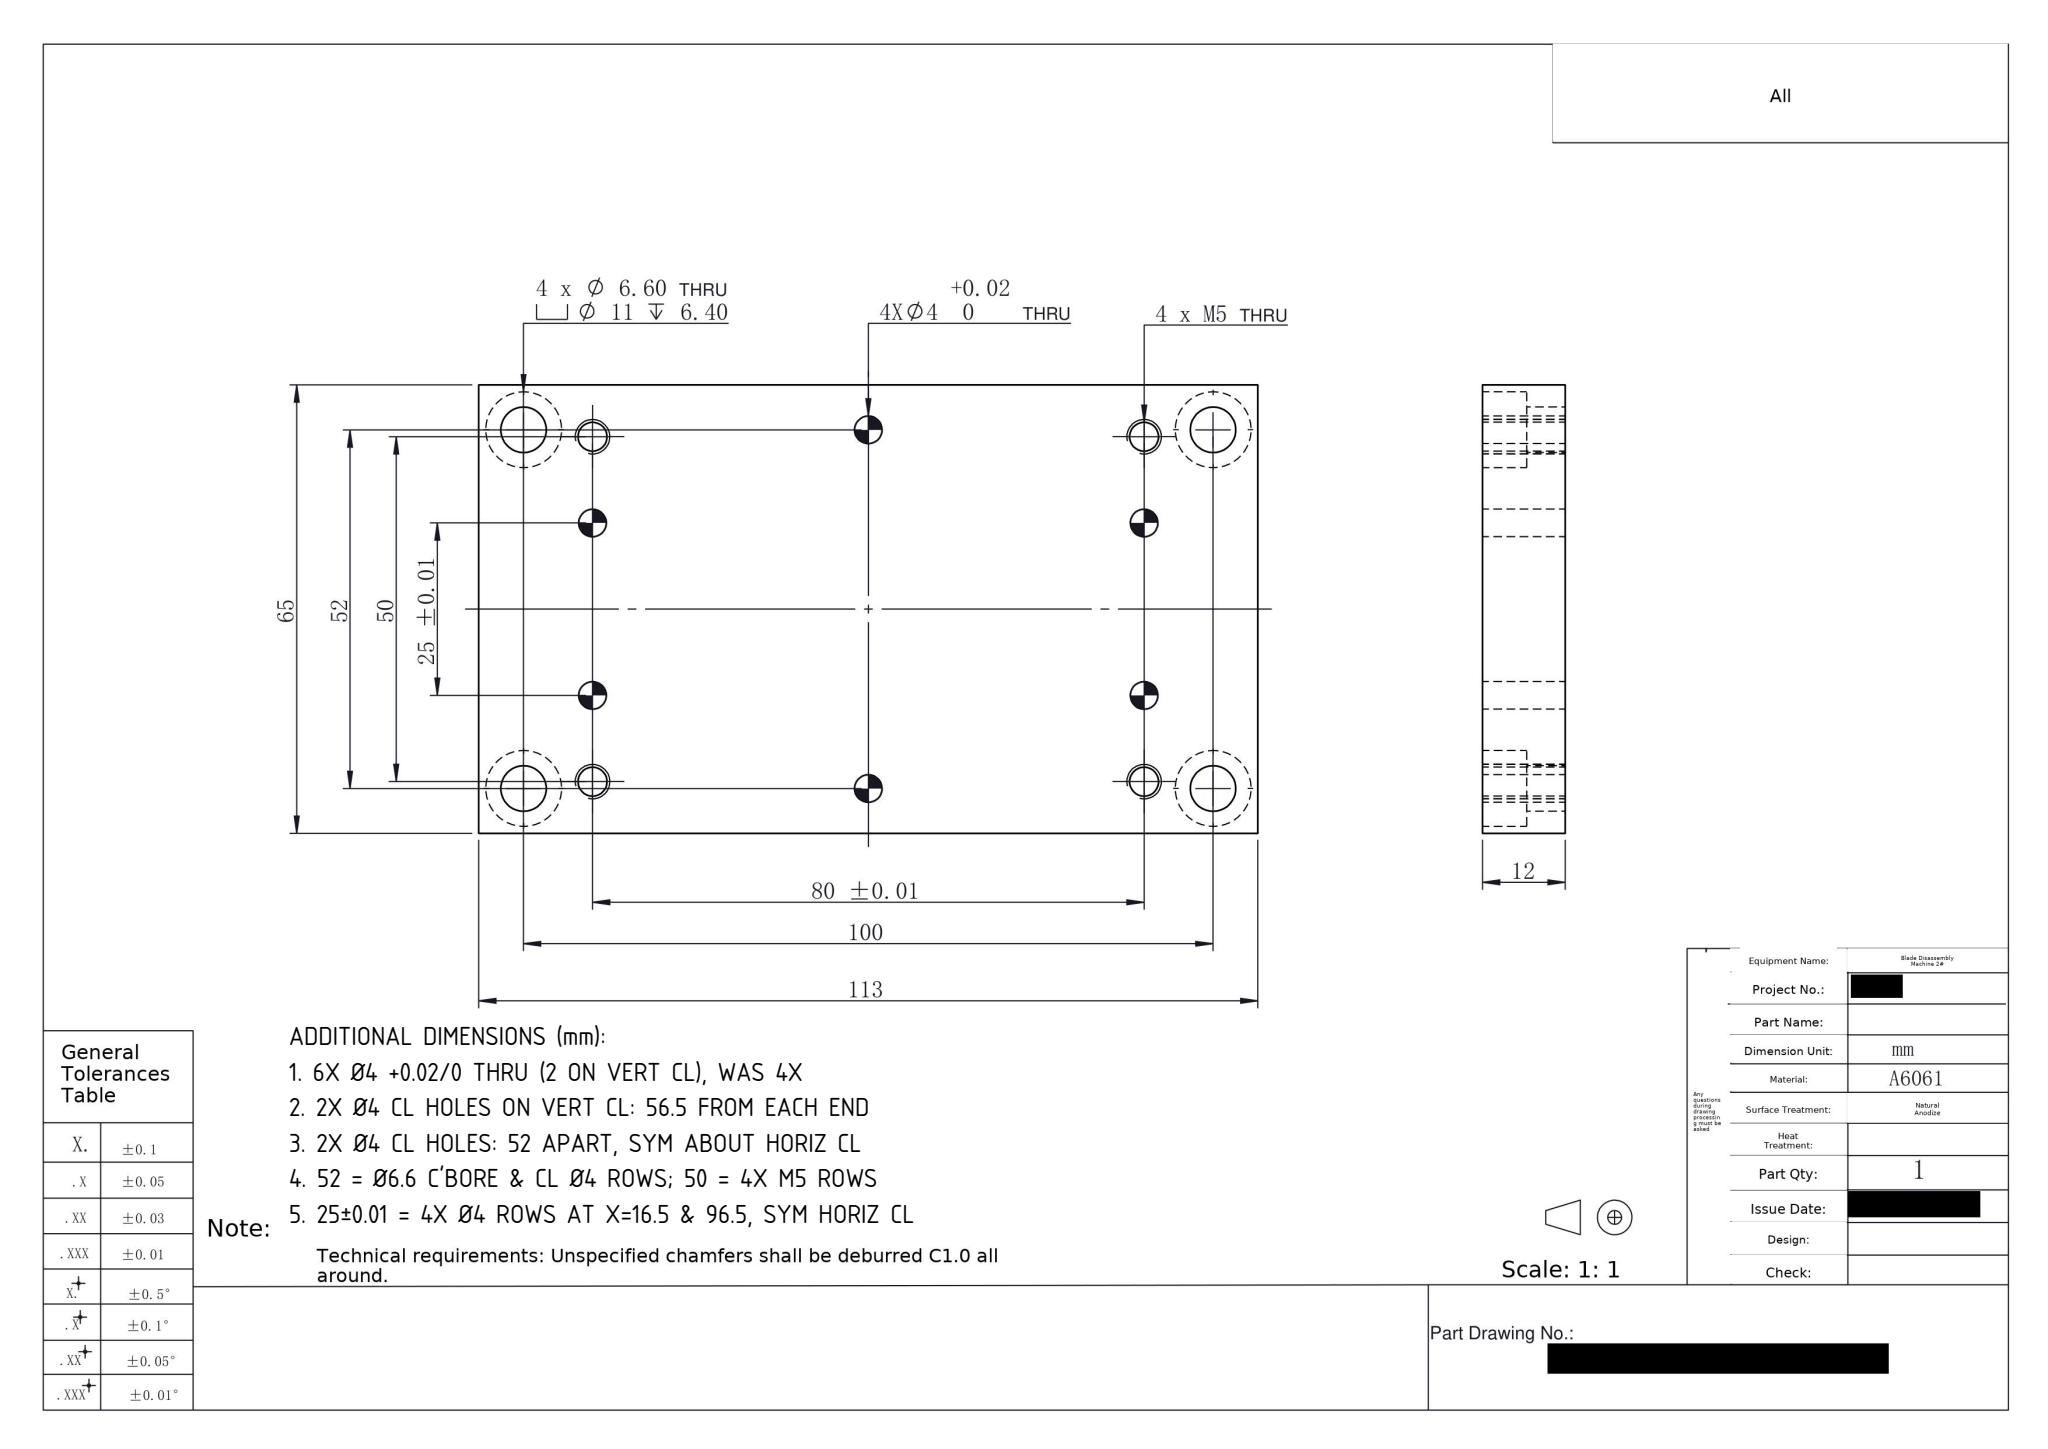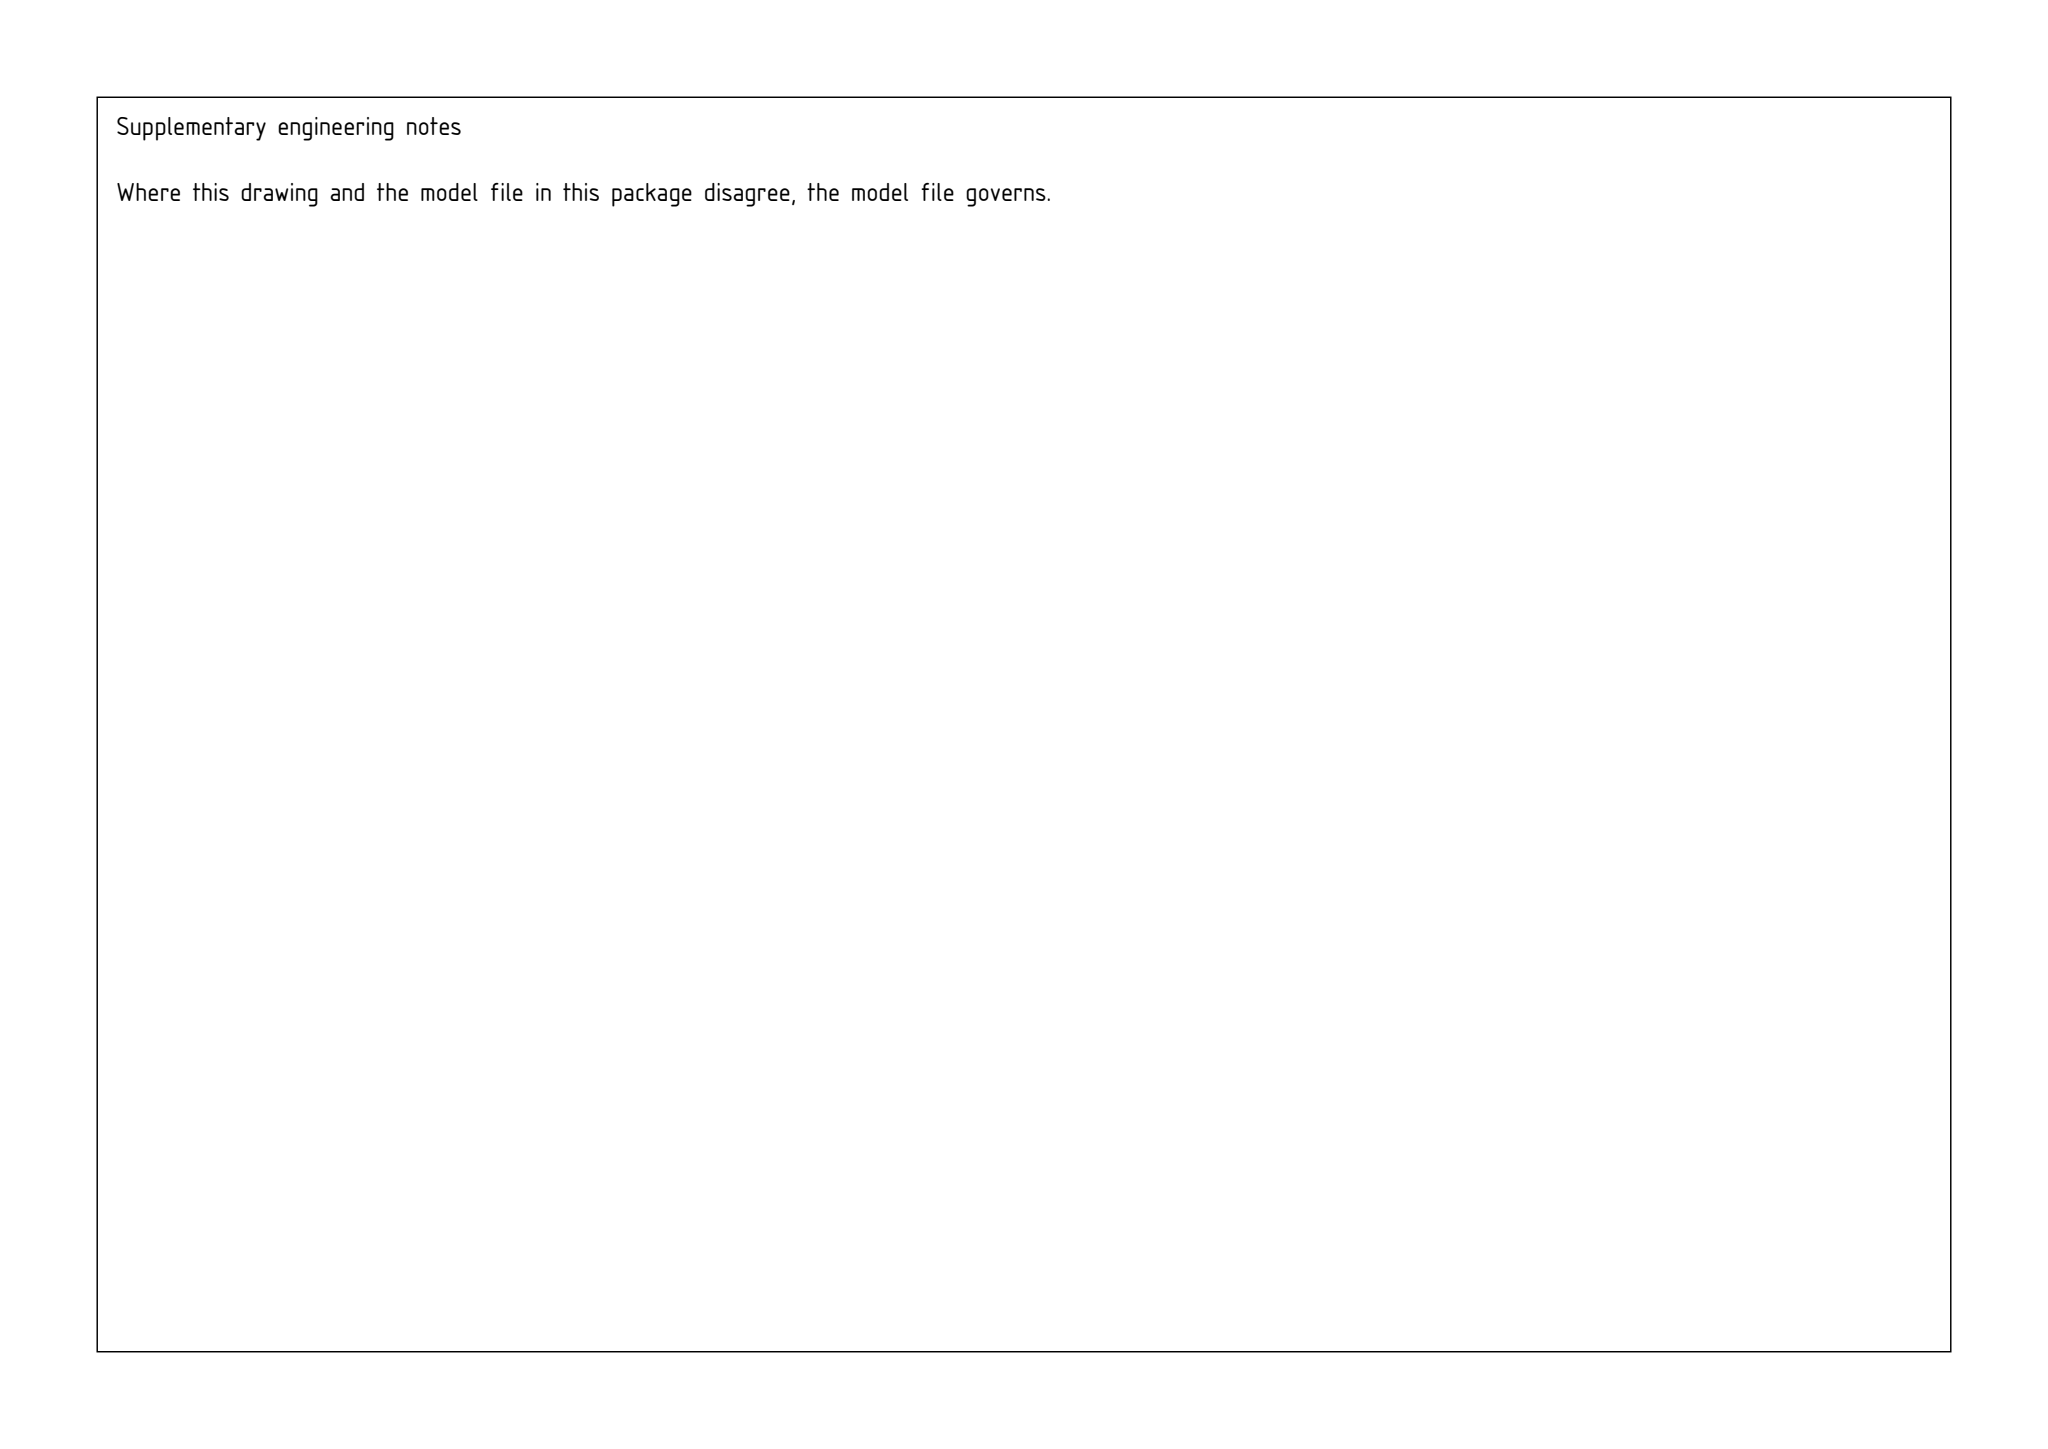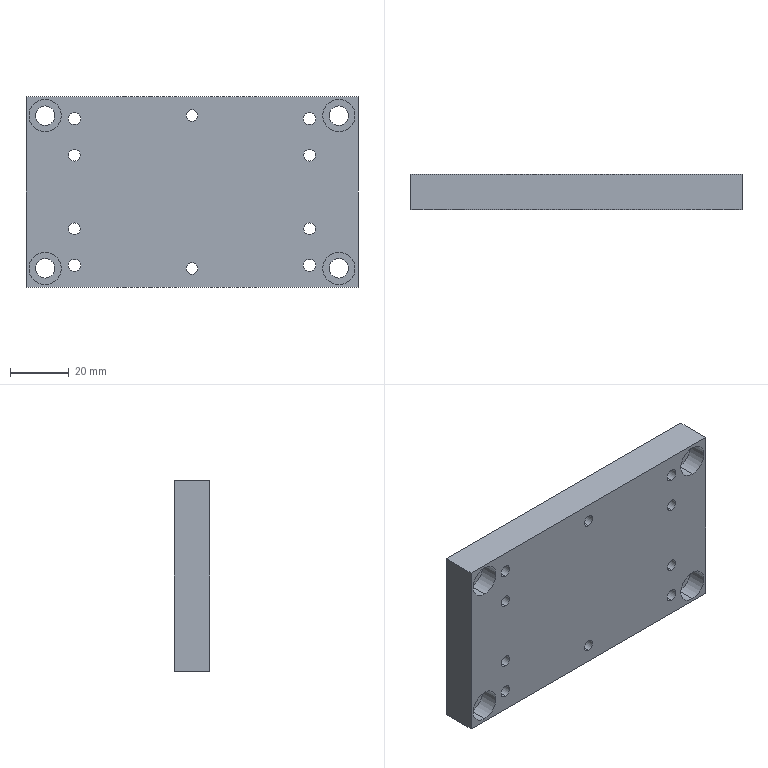Part | SolidWorks | mm | 1 solid | 46 faces | box 113 x 12 x 65 mm | volume 83371 mm3 | cylinder 36 | plane 10 | commonest cylinder face diameters 4 x12 4.2 x8 11 x8 6.6 x8
build123d program:
from build123d import *

# Parameters (mm, degrees)
SKETCH1_W                                       = 113
SKETCH1_H                                       = 65
BOSS_EXTRUDE1_DEPTH                             = 6
M6_HEX_SOCKET_HEAD_CAP_SCREW_CBORE1_D           = 6.6
M6_HEX_SOCKET_HEAD_CAP_SCREW_CBORE1_CBORE_D     = 11
M6_HEX_SOCKET_HEAD_CAP_SCREW_CBORE1_CBORE_DEPTH = 6.4
F_4_0MM_DOWEL_PIN_HOLE1_D                       = 4
M5_TAPPED_HOLE1_D                               = 4.2


with BuildPart() as part:
    # Sketch1 → Boss-Extrude1 (new, symmetric)
    with BuildSketch(Plane(origin=(0, 0, 0), x_dir=(1, 0, 0), z_dir=(0, 1, 0))):
        Rectangle(SKETCH1_W, SKETCH1_H)
    extrude(amount=BOSS_EXTRUDE1_DEPTH, both=True)

    # M6 Hex Socket Head Cap Screw CBORE1 (through all)
    with Locations(Plane(origin=(0, -6, 0), x_dir=(-1, 0, 0), z_dir=(0, -1, 0))):
        with Locations((-50, 26), (-50, -26), (50, -26), (50, 26)):
            CounterBoreHole(M6_HEX_SOCKET_HEAD_CAP_SCREW_CBORE1_D / 2, M6_HEX_SOCKET_HEAD_CAP_SCREW_CBORE1_CBORE_D / 2, M6_HEX_SOCKET_HEAD_CAP_SCREW_CBORE1_CBORE_DEPTH)

    # 4.0mm Dowel Pin Hole1 (through all)
    with Locations(Plane(origin=(0, -6, 0), x_dir=(-1, 0, 0), z_dir=(0, -1, 0))):
        with Locations((0, -26), (0, 26), (-40, -12.5), (40, -12.5), (40, 12.5), (-40, 12.5)):
            Hole(F_4_0MM_DOWEL_PIN_HOLE1_D / 2)

    # M5 Tapped Hole1 (through all)
    with Locations(Plane(origin=(0, -6, 0), x_dir=(-1, 0, 0), z_dir=(0, -1, 0))):
        with Locations((-40, 25), (-40, -25), (40, -25), (40, 25)):
            Hole(M5_TAPPED_HOLE1_D / 2)


solid = part.part